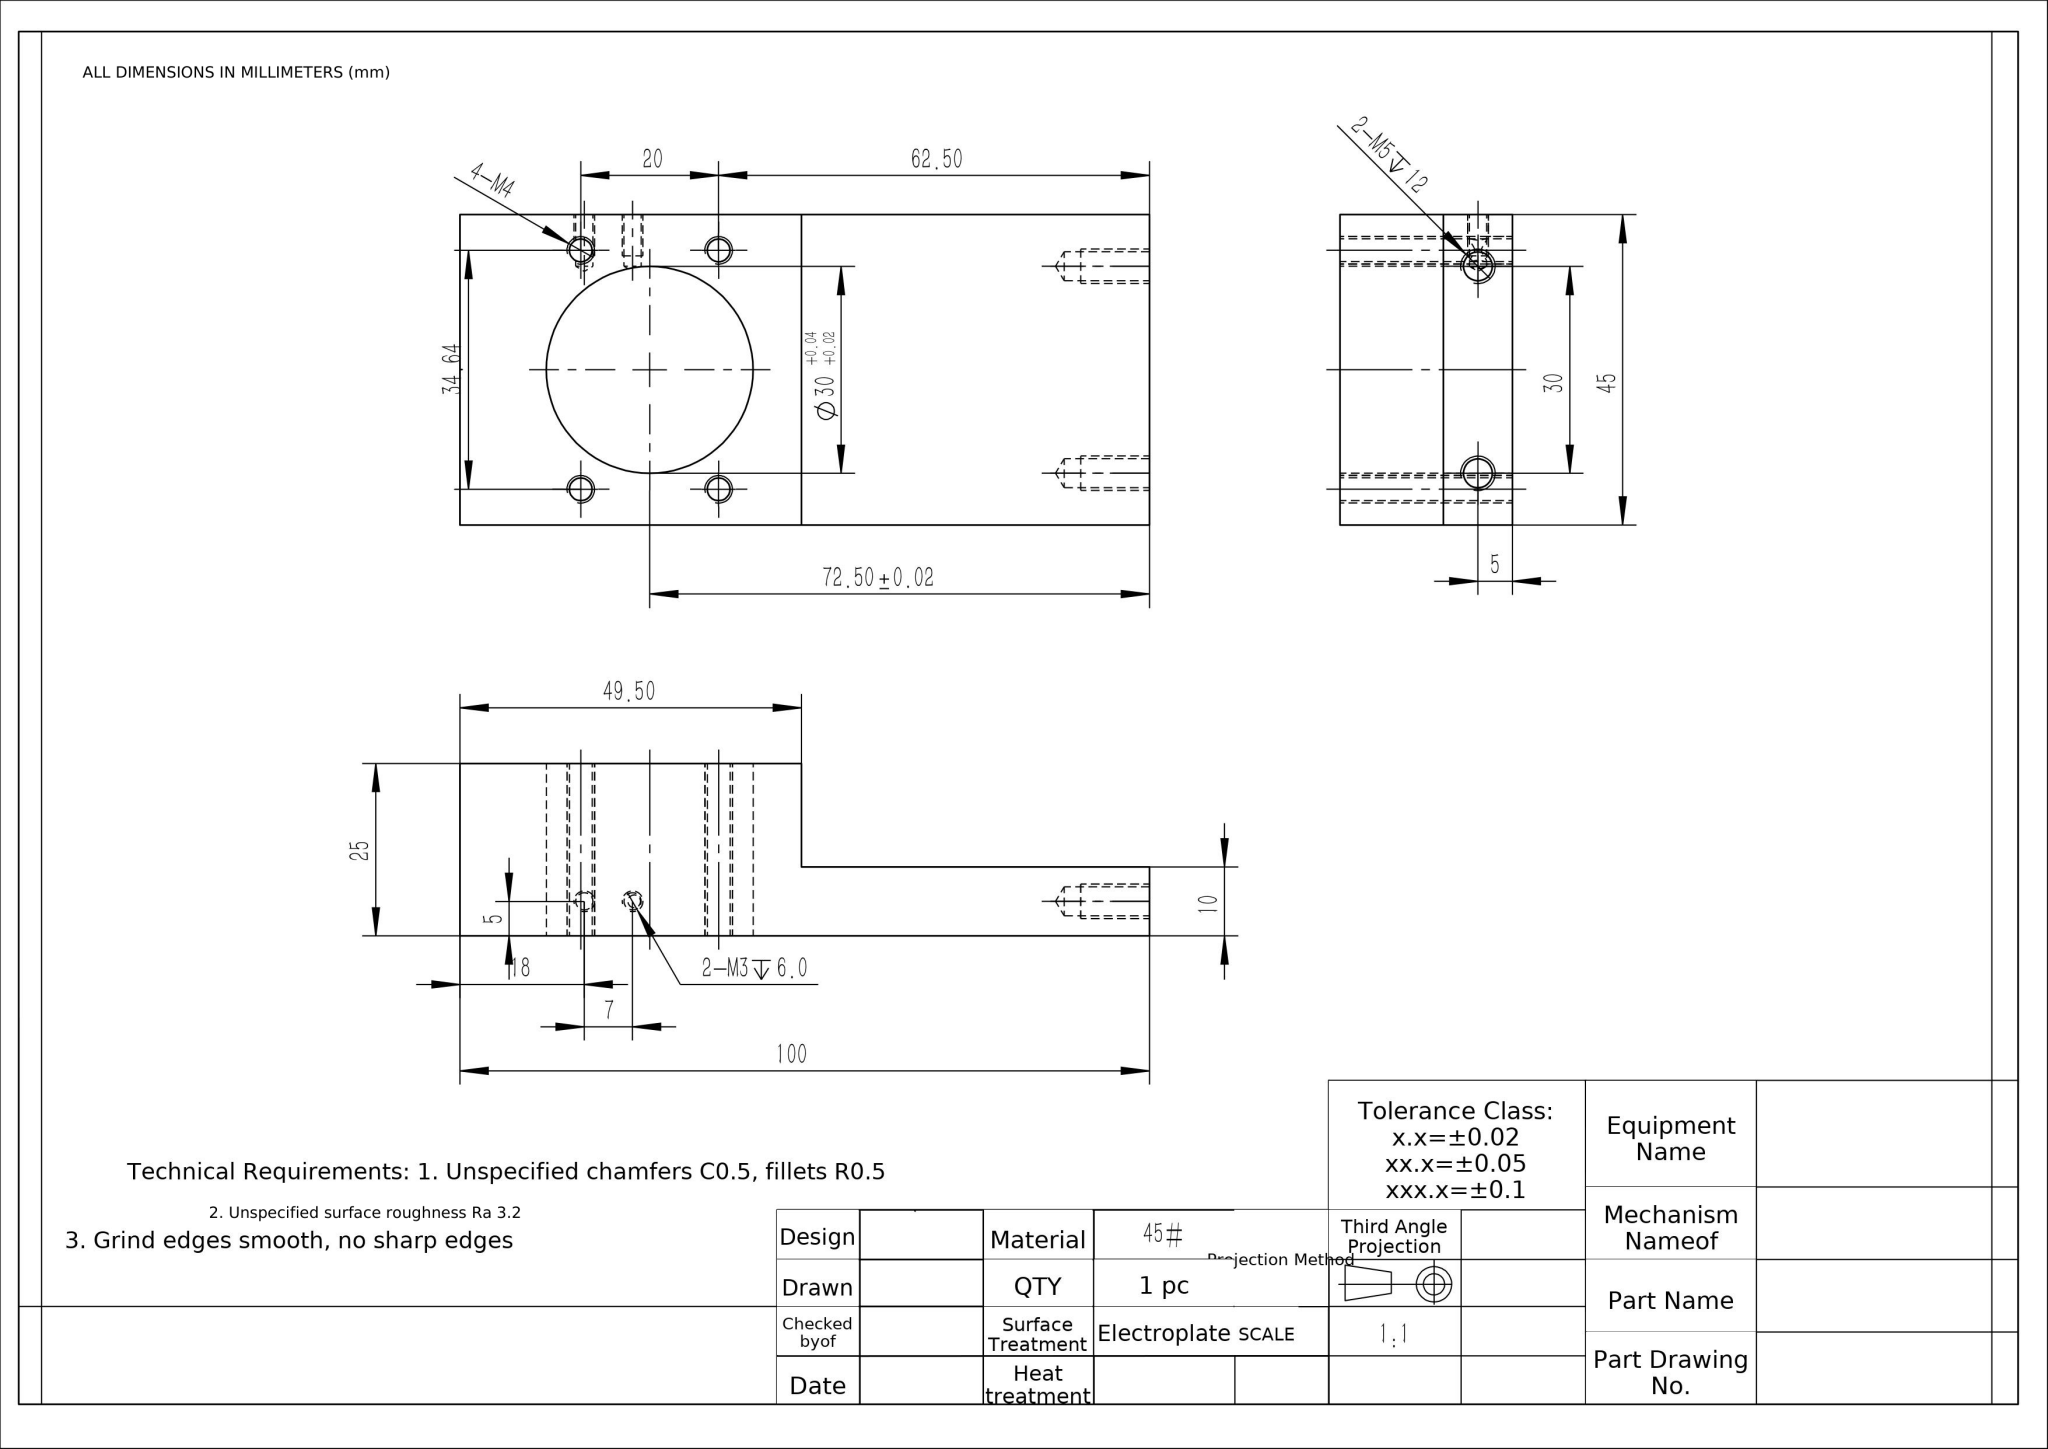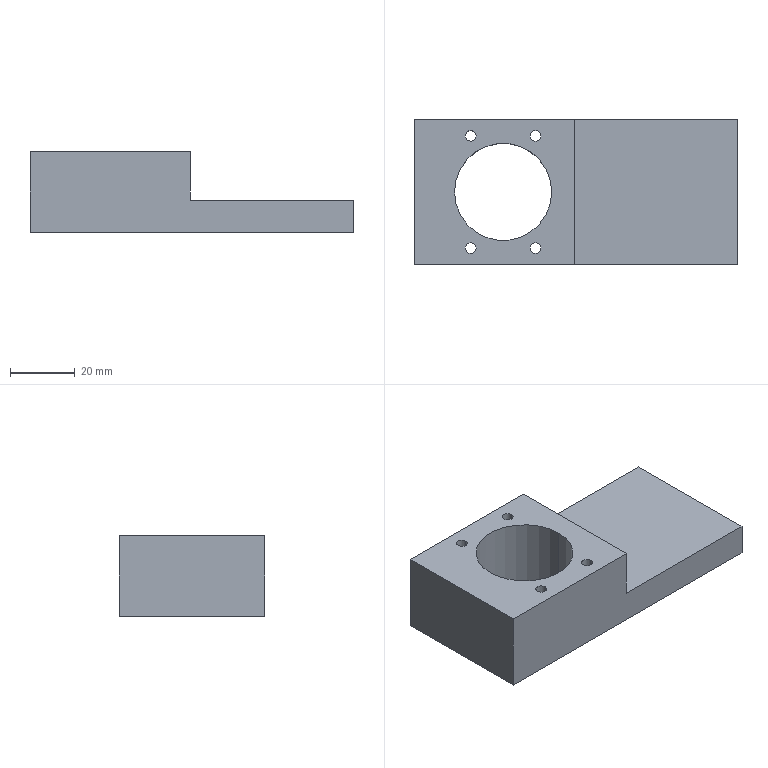Part | NX | mm | 1 solid | 35 faces | box 100 x 45 x 25 mm | volume 59469 mm3 | cylinder 19 | cone 8 | plane 8 | commonest cylinder face diameters 3.3 x8 2.5 x5 4.2 x4 30 x2